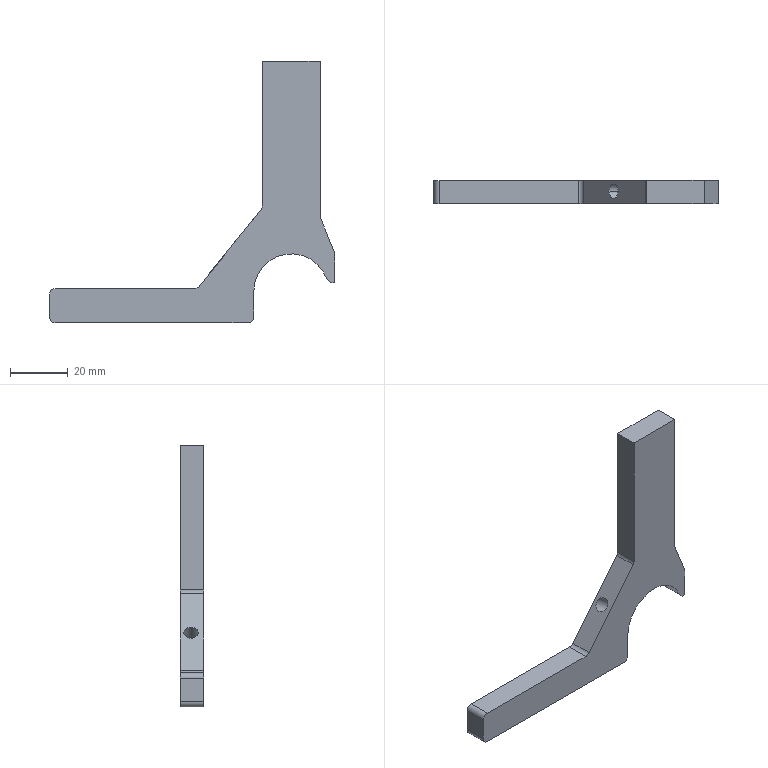Component | SolidWorks | BearingLiftingModule-1_CHEN123-AA-24-1 | 1 solid | 24 faces | box 99 x 8 x 91 mm | volume 20489 mm3 | plane 14 | cylinder 10 | commonest cylinder face diameters 4 x7 5 x2 26.05 x1
STEP:
#1=CARTESIAN_POINT('',(2.27,1.567,1.346));
#2=VERTEX_POINT('',#1);
#3=CARTESIAN_POINT('',(2.37,1.567,1.518));
#4=VERTEX_POINT('',#3);
#5=CARTESIAN_POINT('',(2.27,1.567,1.346));
#6=CARTESIAN_POINT('',(2.27,1.561,1.346));
#7=CARTESIAN_POINT('',(2.27,1.554,1.346));
#8=CARTESIAN_POINT('',(2.271,1.542,1.349));
#9=CARTESIAN_POINT('',(2.272,1.535,1.351));
#10=CARTESIAN_POINT('',(2.274,1.524,1.356));
#11=CARTESIAN_POINT('',(2.275,1.518,1.359));
#12=CARTESIAN_POINT('',(2.278,1.507,1.366));
#13=CARTESIAN_POINT('',(2.279,1.502,1.37));
#14=CARTESIAN_POINT('',(2.283,1.493,1.378));
#15=CARTESIAN_POINT('',(2.285,1.489,1.383));
#16=CARTESIAN_POINT('',(2.289,1.482,1.393));
#17=CARTESIAN_POINT('',(2.291,1.479,1.398));
#18=CARTESIAN_POINT('',(2.299,1.472,1.415));
#19=CARTESIAN_POINT('',(2.305,1.469,1.426));
#20=CARTESIAN_POINT('',(2.315,1.469,1.443));
#21=CARTESIAN_POINT('',(2.318,1.469,1.449));
#22=CARTESIAN_POINT('',(2.325,1.472,1.459));
#23=CARTESIAN_POINT('',(2.329,1.474,1.465));
#24=CARTESIAN_POINT('',(2.335,1.478,1.475));
#25=CARTESIAN_POINT('',(2.339,1.481,1.479));
#26=CARTESIAN_POINT('',(2.345,1.489,1.488));
#27=CARTESIAN_POINT('',(2.348,1.493,1.492));
#28=CARTESIAN_POINT('',(2.357,1.506,1.503));
#29=CARTESIAN_POINT('',(2.361,1.517,1.509));
#30=CARTESIAN_POINT('',(2.366,1.535,1.515));
#31=CARTESIAN_POINT('',(2.368,1.542,1.516));
#32=CARTESIAN_POINT('',(2.369,1.554,1.518));
#33=CARTESIAN_POINT('',(2.37,1.561,1.518));
#34=CARTESIAN_POINT('',(2.37,1.567,1.518));
#35=B_SPLINE_CURVE_WITH_KNOTS('',3,(#5,#6,#7,#8,#9,#10,#11,#12,#13,#14,#15,#16,#17,#18,#19,#20,#21,#22,#23,#24,#25,#26,#27,#28,#29,#30,#31,#32,#33,#34),.UNSPECIFIED.,.F.,.F.,(4,2,2,2,2,2,2,2,2,2,2,2,2,2,4),(0.007885,0.008378,0.008871,0.009363,0.009856,0.01035,0.01084,0.01183,0.01232,0.01281,0.0133,0.0138,0.01478,0.01527,0.01577),.UNSPECIFIED.);
#36=EDGE_CURVE('',#2,#4,#35,.T.);
#37=ORIENTED_EDGE('',*,*,#36,.F.);
#38=CARTESIAN_POINT('',(1.849,1.567,1.687));
#39=VERTEX_POINT('',#38);
#40=CARTESIAN_POINT('',(1.849,1.567,1.687));
#41=DIRECTION('',(-0.7772,0.,0.6292));
#42=VECTOR('',#41,39.37);
#43=LINE('',#40,#42);
#44=EDGE_CURVE('',#2,#39,#43,.T.);
#45=ORIENTED_EDGE('',*,*,#44,.T.);
#46=CARTESIAN_POINT('',(1.973,1.567,1.84));
#47=VERTEX_POINT('',#46);
#48=CARTESIAN_POINT('',(1.911,1.567,1.763));
#49=DIRECTION('',(-0.7772,0.,0.6292));
#50=DIRECTION('',(0.6292,0.,0.7772));
#51=AXIS2_PLACEMENT_3D('',#48,#49,#50);
#52=CIRCLE('',#51,0.09843);
#53=EDGE_CURVE('',#39,#47,#52,.T.);
#54=ORIENTED_EDGE('',*,*,#53,.T.);
#55=CARTESIAN_POINT('',(1.973,1.567,1.84));
#56=DIRECTION('',(-0.7772,0.,0.6292));
#57=VECTOR('',#56,39.37);
#58=LINE('',#55,#57);
#59=EDGE_CURVE('',#4,#47,#58,.T.);
#60=ORIENTED_EDGE('',*,*,#59,.F.);
#61=EDGE_LOOP('',(#37,#45,#54,#60));
#62=FACE_OUTER_BOUND('',#61,.T.);
#63=CARTESIAN_POINT('',(1.911,1.567,1.763));
#64=DIRECTION('',(-0.7772,0.,0.6292));
#65=DIRECTION('',(0.6292,0.,0.7772));
#66=AXIS2_PLACEMENT_3D('',#63,#64,#65);
#67=CYLINDRICAL_SURFACE('',#66,0.09843);
#68=ADVANCED_FACE('',(#62),#67,.F.);
#69=CARTESIAN_POINT('',(2.164,1.713,0.748));
#70=VERTEX_POINT('',#69);
#71=CARTESIAN_POINT('',(-0.4725,1.713,0.748));
#72=VERTEX_POINT('',#71);
#73=CARTESIAN_POINT('',(-0.5512,1.713,0.748));
#74=DIRECTION('',(-1.,0.,0.));
#75=VECTOR('',#74,39.37);
#76=LINE('',#73,#75);
#77=EDGE_CURVE('',#70,#72,#76,.T.);
#78=ORIENTED_EDGE('',*,*,#77,.F.);
#79=CARTESIAN_POINT('',(2.164,1.398,0.748));
#80=VERTEX_POINT('',#79);
#81=CARTESIAN_POINT('',(2.164,1.713,0.748));
#82=DIRECTION('',(0.,-1.,0.));
#83=VECTOR('',#82,39.37);
#84=LINE('',#81,#83);
#85=EDGE_CURVE('',#70,#80,#84,.T.);
#86=ORIENTED_EDGE('',*,*,#85,.T.);
#87=CARTESIAN_POINT('',(-0.4725,1.398,0.748));
#88=VERTEX_POINT('',#87);
#89=CARTESIAN_POINT('',(-0.5512,1.398,0.748));
#90=DIRECTION('',(-1.,0.,0.));
#91=VECTOR('',#90,39.37);
#92=LINE('',#89,#91);
#93=EDGE_CURVE('',#80,#88,#92,.T.);
#94=ORIENTED_EDGE('',*,*,#93,.T.);
#95=CARTESIAN_POINT('',(-0.4725,1.713,0.748));
#96=DIRECTION('',(0.,1.,0.));
#97=VECTOR('',#96,39.37);
#98=LINE('',#95,#97);
#99=EDGE_CURVE('',#88,#72,#98,.T.);
#100=ORIENTED_EDGE('',*,*,#99,.T.);
#101=EDGE_LOOP('',(#78,#86,#94,#100));
#102=FACE_OUTER_BOUND('',#101,.T.);
#103=CARTESIAN_POINT('',(-0.5512,1.713,0.748));
#104=DIRECTION('',(0.,0.,1.));
#105=DIRECTION('',(0.,-1.,0.));
#106=AXIS2_PLACEMENT_3D('',#103,#104,#105);
#107=PLANE('',#106);
#108=ADVANCED_FACE('',(#102),#107,.F.);
#109=CARTESIAN_POINT('',(3.346,1.713,1.695));
#110=VERTEX_POINT('',#109);
#111=CARTESIAN_POINT('',(3.346,1.713,1.299));
#112=VERTEX_POINT('',#111);
#113=CARTESIAN_POINT('',(3.346,1.713,4.331));
#114=DIRECTION('',(0.,0.,-1.));
#115=VECTOR('',#114,39.37);
#116=LINE('',#113,#115);
#117=EDGE_CURVE('',#110,#112,#116,.T.);
#118=ORIENTED_EDGE('',*,*,#117,.F.);
#119=CARTESIAN_POINT('',(3.346,1.398,1.695));
#120=VERTEX_POINT('',#119);
#121=CARTESIAN_POINT('',(3.346,1.713,1.695));
#122=DIRECTION('',(0.,-1.,0.));
#123=VECTOR('',#122,39.37);
#124=LINE('',#121,#123);
#125=EDGE_CURVE('',#110,#120,#124,.T.);
#126=ORIENTED_EDGE('',*,*,#125,.T.);
#127=CARTESIAN_POINT('',(3.346,1.398,1.299));
#128=VERTEX_POINT('',#127);
#129=CARTESIAN_POINT('',(3.346,1.398,4.331));
#130=DIRECTION('',(0.,0.,-1.));
#131=VECTOR('',#130,39.37);
#132=LINE('',#129,#131);
#133=EDGE_CURVE('',#120,#128,#132,.T.);
#134=ORIENTED_EDGE('',*,*,#133,.T.);
#135=CARTESIAN_POINT('',(3.346,1.713,1.299));
#136=DIRECTION('',(0.,1.,0.));
#137=VECTOR('',#136,39.37);
#138=LINE('',#135,#137);
#139=EDGE_CURVE('',#128,#112,#138,.T.);
#140=ORIENTED_EDGE('',*,*,#139,.T.);
#141=EDGE_LOOP('',(#118,#126,#134,#140));
#142=FACE_OUTER_BOUND('',#141,.T.);
#143=CARTESIAN_POINT('',(3.346,1.713,4.331));
#144=DIRECTION('',(-1.,0.,0.));
#145=DIRECTION('',(0.,1.,0.));
#146=AXIS2_PLACEMENT_3D('',#143,#144,#145);
#147=PLANE('',#146);
#148=ADVANCED_FACE('',(#142),#147,.F.);
#149=CARTESIAN_POINT('',(-0.5512,1.713,0.8268));
#150=VERTEX_POINT('',#149);
#151=CARTESIAN_POINT('',(-0.5512,1.713,1.142));
#152=VERTEX_POINT('',#151);
#153=CARTESIAN_POINT('',(-0.5512,1.713,4.331));
#154=DIRECTION('',(0.,0.,1.));
#155=VECTOR('',#154,39.37);
#156=LINE('',#153,#155);
#157=EDGE_CURVE('',#150,#152,#156,.T.);
#158=ORIENTED_EDGE('',*,*,#157,.F.);
#159=CARTESIAN_POINT('',(-0.5512,1.398,0.8268));
#160=VERTEX_POINT('',#159);
#161=CARTESIAN_POINT('',(-0.5512,1.713,0.8268));
#162=DIRECTION('',(0.,-1.,0.));
#163=VECTOR('',#162,39.37);
#164=LINE('',#161,#163);
#165=EDGE_CURVE('',#150,#160,#164,.T.);
#166=ORIENTED_EDGE('',*,*,#165,.T.);
#167=CARTESIAN_POINT('',(-0.5512,1.398,1.142));
#168=VERTEX_POINT('',#167);
#169=CARTESIAN_POINT('',(-0.5512,1.398,4.331));
#170=DIRECTION('',(0.,0.,1.));
#171=VECTOR('',#170,39.37);
#172=LINE('',#169,#171);
#173=EDGE_CURVE('',#160,#168,#172,.T.);
#174=ORIENTED_EDGE('',*,*,#173,.T.);
#175=CARTESIAN_POINT('',(-0.5512,1.713,1.142));
#176=DIRECTION('',(0.,1.,0.));
#177=VECTOR('',#176,39.37);
#178=LINE('',#175,#177);
#179=EDGE_CURVE('',#168,#152,#178,.T.);
#180=ORIENTED_EDGE('',*,*,#179,.T.);
#181=EDGE_LOOP('',(#158,#166,#174,#180));
#182=FACE_OUTER_BOUND('',#181,.T.);
#183=CARTESIAN_POINT('',(-0.5512,1.713,4.331));
#184=DIRECTION('',(1.,0.,0.));
#185=DIRECTION('',(0.,-1.,0.));
#186=AXIS2_PLACEMENT_3D('',#183,#184,#185);
#187=PLANE('',#186);
#188=ADVANCED_FACE('',(#182),#187,.F.);
#189=CARTESIAN_POINT('',(2.362,1.398,4.331));
#190=VERTEX_POINT('',#189);
#191=CARTESIAN_POINT('',(3.15,1.398,4.331));
#192=VERTEX_POINT('',#191);
#193=CARTESIAN_POINT('',(-0.5512,1.398,4.331));
#194=DIRECTION('',(1.,0.,0.));
#195=VECTOR('',#194,39.37);
#196=LINE('',#193,#195);
#197=EDGE_CURVE('',#190,#192,#196,.T.);
#198=ORIENTED_EDGE('',*,*,#197,.T.);
#199=CARTESIAN_POINT('',(3.15,1.713,4.331));
#200=VERTEX_POINT('',#199);
#201=CARTESIAN_POINT('',(3.15,1.398,4.331));
#202=DIRECTION('',(0.,1.,0.));
#203=VECTOR('',#202,39.37);
#204=LINE('',#201,#203);
#205=EDGE_CURVE('',#192,#200,#204,.T.);
#206=ORIENTED_EDGE('',*,*,#205,.T.);
#207=CARTESIAN_POINT('',(2.362,1.713,4.331));
#208=VERTEX_POINT('',#207);
#209=CARTESIAN_POINT('',(-0.5512,1.713,4.331));
#210=DIRECTION('',(1.,0.,0.));
#211=VECTOR('',#210,39.37);
#212=LINE('',#209,#211);
#213=EDGE_CURVE('',#208,#200,#212,.T.);
#214=ORIENTED_EDGE('',*,*,#213,.F.);
#215=CARTESIAN_POINT('',(2.362,1.398,4.331));
#216=DIRECTION('',(0.,1.,0.));
#217=VECTOR('',#216,39.37);
#218=LINE('',#215,#217);
#219=EDGE_CURVE('',#190,#208,#218,.T.);
#220=ORIENTED_EDGE('',*,*,#219,.F.);
#221=EDGE_LOOP('',(#198,#206,#214,#220));
#222=FACE_OUTER_BOUND('',#221,.T.);
#223=CARTESIAN_POINT('',(-0.5512,1.713,4.331));
#224=DIRECTION('',(0.,0.,-1.));
#225=DIRECTION('',(0.,1.,0.));
#226=AXIS2_PLACEMENT_3D('',#223,#224,#225);
#227=PLANE('',#226);
#228=ADVANCED_FACE('',(#222),#227,.F.);
#229=CARTESIAN_POINT('',(3.341,1.713,1.724));
#230=VERTEX_POINT('',#229);
#231=CARTESIAN_POINT('',(3.155,1.713,2.187));
#232=VERTEX_POINT('',#231);
#233=CARTESIAN_POINT('',(3.346,1.713,1.71));
#234=DIRECTION('',(-0.3723,0.,0.9281));
#235=VECTOR('',#234,39.37);
#236=LINE('',#233,#235);
#237=EDGE_CURVE('',#230,#232,#236,.T.);
#238=ORIENTED_EDGE('',*,*,#237,.F.);
#239=CARTESIAN_POINT('',(3.268,1.713,1.695));
#240=DIRECTION('',(0.,1.,0.));
#241=DIRECTION('',(-1.,0.,-0.));
#242=AXIS2_PLACEMENT_3D('',#239,#240,#241);
#243=CIRCLE('',#242,0.07874);
#244=EDGE_CURVE('',#230,#110,#243,.T.);
#245=ORIENTED_EDGE('',*,*,#244,.T.);
#246=ORIENTED_EDGE('',*,*,#117,.T.);
#247=CARTESIAN_POINT('',(3.294,1.713,1.299));
#248=VERTEX_POINT('',#247);
#249=CARTESIAN_POINT('',(2.959,1.713,1.299));
#250=DIRECTION('',(1.,0.,0.));
#251=VECTOR('',#250,39.37);
#252=LINE('',#249,#251);
#253=EDGE_CURVE('',#248,#112,#252,.T.);
#254=ORIENTED_EDGE('',*,*,#253,.F.);
#255=CARTESIAN_POINT('',(3.238,1.713,1.355));
#256=VERTEX_POINT('',#255);
#257=CARTESIAN_POINT('',(3.238,1.713,1.355));
#258=DIRECTION('',(-0.7071,0.,0.7071));
#259=VECTOR('',#258,39.37);
#260=LINE('',#257,#259);
#261=EDGE_CURVE('',#248,#256,#260,.T.);
#262=ORIENTED_EDGE('',*,*,#261,.T.);
#263=CARTESIAN_POINT('',(2.243,1.713,1.181));
#264=VERTEX_POINT('',#263);
#265=CARTESIAN_POINT('',(2.756,1.713,1.181));
#266=DIRECTION('',(0.,1.,0.));
#267=DIRECTION('',(1.,0.,0.));
#268=AXIS2_PLACEMENT_3D('',#265,#266,#267);
#269=CIRCLE('',#268,0.5128);
#270=EDGE_CURVE('',#264,#256,#269,.T.);
#271=ORIENTED_EDGE('',*,*,#270,.F.);
#272=CARTESIAN_POINT('',(2.243,1.713,0.8268));
#273=VERTEX_POINT('',#272);
#274=CARTESIAN_POINT('',(2.243,1.713,1.181));
#275=DIRECTION('',(0.,0.,1.));
#276=VECTOR('',#275,39.37);
#277=LINE('',#274,#276);
#278=EDGE_CURVE('',#273,#264,#277,.T.);
#279=ORIENTED_EDGE('',*,*,#278,.F.);
#280=CARTESIAN_POINT('',(2.164,1.713,0.8268));
#281=DIRECTION('',(0.,1.,0.));
#282=DIRECTION('',(-1.,0.,0.));
#283=AXIS2_PLACEMENT_3D('',#280,#281,#282);
#284=CIRCLE('',#283,0.07874);
#285=EDGE_CURVE('',#273,#70,#284,.T.);
#286=ORIENTED_EDGE('',*,*,#285,.T.);
#287=ORIENTED_EDGE('',*,*,#77,.T.);
#288=CARTESIAN_POINT('',(-0.4725,1.713,0.8268));
#289=DIRECTION('',(0.,1.,0.));
#290=DIRECTION('',(-1.,0.,0.));
#291=AXIS2_PLACEMENT_3D('',#288,#289,#290);
#292=CIRCLE('',#291,0.07874);
#293=EDGE_CURVE('',#72,#150,#292,.T.);
#294=ORIENTED_EDGE('',*,*,#293,.T.);
#295=ORIENTED_EDGE('',*,*,#157,.T.);
#296=CARTESIAN_POINT('',(-0.4725,1.713,1.22));
#297=VERTEX_POINT('',#296);
#298=CARTESIAN_POINT('',(-0.4725,1.713,1.142));
#299=DIRECTION('',(0.,1.,0.));
#300=DIRECTION('',(-1.,0.,0.));
#301=AXIS2_PLACEMENT_3D('',#298,#299,#300);
#302=CIRCLE('',#301,0.07874);
#303=EDGE_CURVE('',#152,#297,#302,.T.);
#304=ORIENTED_EDGE('',*,*,#303,.T.);
#305=CARTESIAN_POINT('',(1.434,1.713,1.22));
#306=VERTEX_POINT('',#305);
#307=CARTESIAN_POINT('',(-0.5512,1.713,1.22));
#308=DIRECTION('',(-1.,0.,0.));
#309=VECTOR('',#308,39.37);
#310=LINE('',#307,#309);
#311=EDGE_CURVE('',#306,#297,#310,.T.);
#312=ORIENTED_EDGE('',*,*,#311,.F.);
#313=CARTESIAN_POINT('',(1.495,1.713,1.25));
#314=VERTEX_POINT('',#313);
#315=CARTESIAN_POINT('',(1.434,1.713,1.299));
#316=DIRECTION('',(0.,-1.,0.));
#317=DIRECTION('',(-1.,0.,0.));
#318=AXIS2_PLACEMENT_3D('',#315,#316,#317);
#319=CIRCLE('',#318,0.07874);
#320=EDGE_CURVE('',#306,#314,#319,.T.);
#321=ORIENTED_EDGE('',*,*,#320,.T.);
#322=CARTESIAN_POINT('',(2.345,1.713,2.299));
#323=VERTEX_POINT('',#322);
#324=CARTESIAN_POINT('',(1.471,1.713,1.22));
#325=DIRECTION('',(-0.6292,0.,-0.7772));
#326=VECTOR('',#325,39.37);
#327=LINE('',#324,#326);
#328=EDGE_CURVE('',#323,#314,#327,.T.);
#329=ORIENTED_EDGE('',*,*,#328,.F.);
#330=CARTESIAN_POINT('',(2.362,1.713,2.349));
#331=VERTEX_POINT('',#330);
#332=CARTESIAN_POINT('',(2.283,1.713,2.349));
#333=DIRECTION('',(0.,-1.,0.));
#334=DIRECTION('',(-1.,0.,0.));
#335=AXIS2_PLACEMENT_3D('',#332,#333,#334);
#336=CIRCLE('',#335,0.07874);
#337=EDGE_CURVE('',#323,#331,#336,.T.);
#338=ORIENTED_EDGE('',*,*,#337,.T.);
#339=CARTESIAN_POINT('',(2.362,1.713,2.321));
#340=DIRECTION('',(-0.,0.,-1.));
#341=VECTOR('',#340,39.37);
#342=LINE('',#339,#341);
#343=EDGE_CURVE('',#208,#331,#342,.T.);
#344=ORIENTED_EDGE('',*,*,#343,.F.);
#345=ORIENTED_EDGE('',*,*,#213,.T.);
#346=CARTESIAN_POINT('',(3.15,1.713,2.216));
#347=VERTEX_POINT('',#346);
#348=CARTESIAN_POINT('',(3.15,1.713,4.331));
#349=DIRECTION('',(0.,0.,1.));
#350=VECTOR('',#349,39.37);
#351=LINE('',#348,#350);
#352=EDGE_CURVE('',#347,#200,#351,.T.);
#353=ORIENTED_EDGE('',*,*,#352,.F.);
#354=CARTESIAN_POINT('',(3.228,1.713,2.216));
#355=DIRECTION('',(0.,-1.,0.));
#356=DIRECTION('',(-1.,0.,0.));
#357=AXIS2_PLACEMENT_3D('',#354,#355,#356);
#358=CIRCLE('',#357,0.07874);
#359=EDGE_CURVE('',#347,#232,#358,.T.);
#360=ORIENTED_EDGE('',*,*,#359,.T.);
#361=EDGE_LOOP('',(#238,#245,#246,#254,#262,#271,#279,#286,#287,#294,#295,#304,#312,#321,#329,#338,#344,#345,#353,#360));
#362=FACE_OUTER_BOUND('',#361,.T.);
#363=CARTESIAN_POINT('',(1.398,1.713,2.539));
#364=DIRECTION('',(0.,-1.,0.));
#365=DIRECTION('',(-1.,0.,0.));
#366=AXIS2_PLACEMENT_3D('',#363,#364,#365);
#367=PLANE('',#366);
#368=ADVANCED_FACE('',(#362),#367,.F.);
#369=ORIENTED_EDGE('',*,*,#133,.F.);
#370=CARTESIAN_POINT('',(3.341,1.398,1.724));
#371=VERTEX_POINT('',#370);
#372=CARTESIAN_POINT('',(3.268,1.398,1.695));
#373=DIRECTION('',(0.,-1.,0.));
#374=DIRECTION('',(-1.,0.,0.));
#375=AXIS2_PLACEMENT_3D('',#372,#373,#374);
#376=CIRCLE('',#375,0.07874);
#377=EDGE_CURVE('',#120,#371,#376,.T.);
#378=ORIENTED_EDGE('',*,*,#377,.T.);
#379=CARTESIAN_POINT('',(3.155,1.398,2.187));
#380=VERTEX_POINT('',#379);
#381=CARTESIAN_POINT('',(3.346,1.398,1.71));
#382=DIRECTION('',(-0.3723,0.,0.9281));
#383=VECTOR('',#382,39.37);
#384=LINE('',#381,#383);
#385=EDGE_CURVE('',#371,#380,#384,.T.);
#386=ORIENTED_EDGE('',*,*,#385,.T.);
#387=CARTESIAN_POINT('',(3.15,1.398,2.216));
#388=VERTEX_POINT('',#387);
#389=CARTESIAN_POINT('',(3.228,1.398,2.216));
#390=DIRECTION('',(0.,1.,0.));
#391=DIRECTION('',(-1.,0.,-0.));
#392=AXIS2_PLACEMENT_3D('',#389,#390,#391);
#393=CIRCLE('',#392,0.07874);
#394=EDGE_CURVE('',#380,#388,#393,.T.);
#395=ORIENTED_EDGE('',*,*,#394,.T.);
#396=CARTESIAN_POINT('',(3.15,1.398,4.331));
#397=DIRECTION('',(0.,0.,1.));
#398=VECTOR('',#397,39.37);
#399=LINE('',#396,#398);
#400=EDGE_CURVE('',#388,#192,#399,.T.);
#401=ORIENTED_EDGE('',*,*,#400,.T.);
#402=ORIENTED_EDGE('',*,*,#197,.F.);
#403=CARTESIAN_POINT('',(2.362,1.398,2.349));
#404=VERTEX_POINT('',#403);
#405=CARTESIAN_POINT('',(2.362,1.398,2.321));
#406=DIRECTION('',(-0.,0.,-1.));
#407=VECTOR('',#406,39.37);
#408=LINE('',#405,#407);
#409=EDGE_CURVE('',#190,#404,#408,.T.);
#410=ORIENTED_EDGE('',*,*,#409,.T.);
#411=CARTESIAN_POINT('',(2.345,1.398,2.299));
#412=VERTEX_POINT('',#411);
#413=CARTESIAN_POINT('',(2.283,1.398,2.349));
#414=DIRECTION('',(0.,1.,0.));
#415=DIRECTION('',(-1.,0.,0.));
#416=AXIS2_PLACEMENT_3D('',#413,#414,#415);
#417=CIRCLE('',#416,0.07874);
#418=EDGE_CURVE('',#404,#412,#417,.T.);
#419=ORIENTED_EDGE('',*,*,#418,.T.);
#420=CARTESIAN_POINT('',(1.495,1.398,1.25));
#421=VERTEX_POINT('',#420);
#422=CARTESIAN_POINT('',(1.471,1.398,1.22));
#423=DIRECTION('',(-0.6292,0.,-0.7772));
#424=VECTOR('',#423,39.37);
#425=LINE('',#422,#424);
#426=EDGE_CURVE('',#412,#421,#425,.T.);
#427=ORIENTED_EDGE('',*,*,#426,.T.);
#428=CARTESIAN_POINT('',(1.434,1.398,1.22));
#429=VERTEX_POINT('',#428);
#430=CARTESIAN_POINT('',(1.434,1.398,1.299));
#431=DIRECTION('',(0.,1.,0.));
#432=DIRECTION('',(-1.,0.,0.));
#433=AXIS2_PLACEMENT_3D('',#430,#431,#432);
#434=CIRCLE('',#433,0.07874);
#435=EDGE_CURVE('',#421,#429,#434,.T.);
#436=ORIENTED_EDGE('',*,*,#435,.T.);
#437=CARTESIAN_POINT('',(-0.4725,1.398,1.22));
#438=VERTEX_POINT('',#437);
#439=CARTESIAN_POINT('',(-0.5512,1.398,1.22));
#440=DIRECTION('',(-1.,0.,0.));
#441=VECTOR('',#440,39.37);
#442=LINE('',#439,#441);
#443=EDGE_CURVE('',#429,#438,#442,.T.);
#444=ORIENTED_EDGE('',*,*,#443,.T.);
#445=CARTESIAN_POINT('',(-0.4725,1.398,1.142));
#446=DIRECTION('',(0.,-1.,0.));
#447=DIRECTION('',(-1.,0.,0.));
#448=AXIS2_PLACEMENT_3D('',#445,#446,#447);
#449=CIRCLE('',#448,0.07874);
#450=EDGE_CURVE('',#438,#168,#449,.T.);
#451=ORIENTED_EDGE('',*,*,#450,.T.);
#452=ORIENTED_EDGE('',*,*,#173,.F.);
#453=CARTESIAN_POINT('',(-0.4725,1.398,0.8268));
#454=DIRECTION('',(0.,-1.,0.));
#455=DIRECTION('',(-1.,0.,0.));
#456=AXIS2_PLACEMENT_3D('',#453,#454,#455);
#457=CIRCLE('',#456,0.07874);
#458=EDGE_CURVE('',#160,#88,#457,.T.);
#459=ORIENTED_EDGE('',*,*,#458,.T.);
#460=ORIENTED_EDGE('',*,*,#93,.F.);
#461=CARTESIAN_POINT('',(2.243,1.398,0.8268));
#462=VERTEX_POINT('',#461);
#463=CARTESIAN_POINT('',(2.164,1.398,0.8268));
#464=DIRECTION('',(0.,-1.,0.));
#465=DIRECTION('',(-1.,0.,0.));
#466=AXIS2_PLACEMENT_3D('',#463,#464,#465);
#467=CIRCLE('',#466,0.07874);
#468=EDGE_CURVE('',#80,#462,#467,.T.);
#469=ORIENTED_EDGE('',*,*,#468,.T.);
#470=CARTESIAN_POINT('',(2.243,1.398,1.181));
#471=VERTEX_POINT('',#470);
#472=CARTESIAN_POINT('',(2.243,1.398,2.539));
#473=DIRECTION('',(0.,0.,-1.));
#474=VECTOR('',#473,39.37);
#475=LINE('',#472,#474);
#476=EDGE_CURVE('',#471,#462,#475,.T.);
#477=ORIENTED_EDGE('',*,*,#476,.F.);
#478=CARTESIAN_POINT('',(3.238,1.398,1.355));
#479=VERTEX_POINT('',#478);
#480=CARTESIAN_POINT('',(2.756,1.398,1.181));
#481=DIRECTION('',(0.,1.,0.));
#482=DIRECTION('',(1.,0.,0.));
#483=AXIS2_PLACEMENT_3D('',#480,#481,#482);
#484=CIRCLE('',#483,0.5128);
#485=EDGE_CURVE('',#471,#479,#484,.T.);
#486=ORIENTED_EDGE('',*,*,#485,.T.);
#487=CARTESIAN_POINT('',(3.294,1.398,1.299));
#488=VERTEX_POINT('',#487);
#489=CARTESIAN_POINT('',(1.726,1.398,2.868));
#490=DIRECTION('',(0.7071,0.,-0.7071));
#491=VECTOR('',#490,39.37);
#492=LINE('',#489,#491);
#493=EDGE_CURVE('',#479,#488,#492,.T.);
#494=ORIENTED_EDGE('',*,*,#493,.T.);
#495=CARTESIAN_POINT('',(2.959,1.398,1.299));
#496=DIRECTION('',(1.,0.,0.));
#497=VECTOR('',#496,39.37);
#498=LINE('',#495,#497);
#499=EDGE_CURVE('',#488,#128,#498,.T.);
#500=ORIENTED_EDGE('',*,*,#499,.T.);
#501=EDGE_LOOP('',(#369,#378,#386,#395,#401,#402,#410,#419,#427,#436,#444,#451,#452,#459,#460,#469,#477,#486,#494,#500));
#502=FACE_OUTER_BOUND('',#501,.T.);
#503=CARTESIAN_POINT('',(1.398,1.398,2.539));
#504=DIRECTION('',(0.,-1.,0.));
#505=DIRECTION('',(-1.,0.,0.));
#506=AXIS2_PLACEMENT_3D('',#503,#504,#505);
#507=PLANE('',#506);
#508=ADVANCED_FACE('',(#502),#507,.T.);
#509=ORIENTED_EDGE('',*,*,#443,.F.);
#510=CARTESIAN_POINT('',(1.434,1.713,1.22));
#511=DIRECTION('',(0.,1.,0.));
#512=VECTOR('',#511,39.37);
#513=LINE('',#510,#512);
#514=EDGE_CURVE('',#429,#306,#513,.T.);
#515=ORIENTED_EDGE('',*,*,#514,.T.);
#516=ORIENTED_EDGE('',*,*,#311,.T.);
#517=CARTESIAN_POINT('',(-0.4725,1.398,1.22));
#518=DIRECTION('',(0.,-1.,0.));
#519=VECTOR('',#518,39.37);
#520=LINE('',#517,#519);
#521=EDGE_CURVE('',#297,#438,#520,.T.);
#522=ORIENTED_EDGE('',*,*,#521,.T.);
#523=EDGE_LOOP('',(#509,#515,#516,#522));
#524=FACE_OUTER_BOUND('',#523,.T.);
#525=CARTESIAN_POINT('',(-0.5512,1.398,1.22));
#526=DIRECTION('',(0.,0.,-1.));
#527=DIRECTION('',(0.,1.,0.));
#528=AXIS2_PLACEMENT_3D('',#525,#526,#527);
#529=PLANE('',#528);
#530=ADVANCED_FACE('',(#524),#529,.F.);
#531=CARTESIAN_POINT('',(1.911,1.567,1.763));
#532=DIRECTION('',(-0.7772,0.,0.6292));
#533=DIRECTION('',(0.6292,0.,0.7772));
#534=AXIS2_PLACEMENT_3D('',#531,#532,#533);
#535=CIRCLE('',#534,0.09843);
#536=EDGE_CURVE('',#47,#39,#535,.T.);
#537=ORIENTED_EDGE('',*,*,#536,.F.);
#538=ORIENTED_EDGE('',*,*,#53,.F.);
#539=EDGE_LOOP('',(#537,#538));
#540=FACE_BOUND('',#539,.T.);
#541=ORIENTED_EDGE('',*,*,#328,.T.);
#542=CARTESIAN_POINT('',(1.495,1.398,1.25));
#543=DIRECTION('',(0.,-1.,0.));
#544=VECTOR('',#543,39.37);
#545=LINE('',#542,#544);
#546=EDGE_CURVE('',#314,#421,#545,.T.);
#547=ORIENTED_EDGE('',*,*,#546,.T.);
#548=ORIENTED_EDGE('',*,*,#426,.F.);
#549=CARTESIAN_POINT('',(2.345,1.713,2.299));
#550=DIRECTION('',(0.,1.,0.));
#551=VECTOR('',#550,39.37);
#552=LINE('',#549,#551);
#553=EDGE_CURVE('',#412,#323,#552,.T.);
#554=ORIENTED_EDGE('',*,*,#553,.T.);
#555=EDGE_LOOP('',(#541,#547,#548,#554));
#556=FACE_OUTER_BOUND('',#555,.T.);
#557=CARTESIAN_POINT('',(1.471,1.398,1.22));
#558=DIRECTION('',(0.7772,0.,-0.6292));
#559=DIRECTION('',(-0.6292,0.,-0.7772));
#560=AXIS2_PLACEMENT_3D('',#557,#558,#559);
#561=PLANE('',#560);
#562=ADVANCED_FACE('',(#540,#556),#561,.F.);
#563=ORIENTED_EDGE('',*,*,#343,.T.);
#564=CARTESIAN_POINT('',(2.362,1.398,2.349));
#565=DIRECTION('',(0.,-1.,0.));
#566=VECTOR('',#565,39.37);
#567=LINE('',#564,#566);
#568=EDGE_CURVE('',#331,#404,#567,.T.);
#569=ORIENTED_EDGE('',*,*,#568,.T.);
#570=ORIENTED_EDGE('',*,*,#409,.F.);
#571=ORIENTED_EDGE('',*,*,#219,.T.);
#572=EDGE_LOOP('',(#563,#569,#570,#571));
#573=FACE_OUTER_BOUND('',#572,.T.);
#574=CARTESIAN_POINT('',(2.362,1.398,2.321));
#575=DIRECTION('',(1.,0.,-0.));
#576=DIRECTION('',(-0.,0.,-1.));
#577=AXIS2_PLACEMENT_3D('',#574,#575,#576);
#578=PLANE('',#577);
#579=ADVANCED_FACE('',(#573),#578,.F.);
#580=ORIENTED_EDGE('',*,*,#476,.T.);
#581=CARTESIAN_POINT('',(2.243,1.398,0.8268));
#582=DIRECTION('',(0.,1.,0.));
#583=VECTOR('',#582,39.37);
#584=LINE('',#581,#583);
#585=EDGE_CURVE('',#462,#273,#584,.T.);
#586=ORIENTED_EDGE('',*,*,#585,.T.);
#587=ORIENTED_EDGE('',*,*,#278,.T.);
#588=CARTESIAN_POINT('',(2.243,1.398,1.181));
#589=DIRECTION('',(0.,1.,0.));
#590=VECTOR('',#589,39.37);
#591=LINE('',#588,#590);
#592=EDGE_CURVE('',#471,#264,#591,.T.);
#593=ORIENTED_EDGE('',*,*,#592,.F.);
#594=EDGE_LOOP('',(#580,#586,#587,#593));
#595=FACE_OUTER_BOUND('',#594,.T.);
#596=CARTESIAN_POINT('',(2.243,1.398,1.181));
#597=DIRECTION('',(-1.,0.,0.));
#598=DIRECTION('',(0.,1.,0.));
#599=AXIS2_PLACEMENT_3D('',#596,#597,#598);
#600=PLANE('',#599);
#601=ADVANCED_FACE('',(#595),#600,.F.);
#602=CARTESIAN_POINT('',(2.37,1.567,1.518));
#603=CARTESIAN_POINT('',(2.37,1.574,1.518));
#604=CARTESIAN_POINT('',(2.369,1.58,1.518));
#605=CARTESIAN_POINT('',(2.368,1.593,1.516));
#606=CARTESIAN_POINT('',(2.366,1.599,1.515));
#607=CARTESIAN_POINT('',(2.363,1.611,1.511));
#608=CARTESIAN_POINT('',(2.361,1.617,1.508));
#609=CARTESIAN_POINT('',(2.357,1.628,1.503));
#610=CARTESIAN_POINT('',(2.354,1.633,1.499));
#611=CARTESIAN_POINT('',(2.348,1.642,1.492));
#612=CARTESIAN_POINT('',(2.345,1.646,1.488));
#613=CARTESIAN_POINT('',(2.339,1.653,1.479));
#614=CARTESIAN_POINT('',(2.335,1.656,1.475));
#615=CARTESIAN_POINT('',(2.329,1.661,1.465));
#616=CARTESIAN_POINT('',(2.325,1.663,1.459));
#617=CARTESIAN_POINT('',(2.318,1.665,1.449));
#618=CARTESIAN_POINT('',(2.315,1.666,1.443));
#619=CARTESIAN_POINT('',(2.309,1.666,1.432));
#620=CARTESIAN_POINT('',(2.305,1.665,1.426));
#621=CARTESIAN_POINT('',(2.299,1.662,1.415));
#622=CARTESIAN_POINT('',(2.297,1.661,1.409));
#623=CARTESIAN_POINT('',(2.291,1.656,1.398));
#624=CARTESIAN_POINT('',(2.289,1.653,1.393));
#625=CARTESIAN_POINT('',(2.285,1.645,1.383));
#626=CARTESIAN_POINT('',(2.283,1.641,1.379));
#627=CARTESIAN_POINT('',(2.279,1.632,1.37));
#628=CARTESIAN_POINT('',(2.278,1.627,1.366));
#629=CARTESIAN_POINT('',(2.275,1.617,1.359));
#630=CARTESIAN_POINT('',(2.274,1.611,1.356));
#631=CARTESIAN_POINT('',(2.272,1.599,1.351));
#632=CARTESIAN_POINT('',(2.271,1.593,1.349));
#633=CARTESIAN_POINT('',(2.27,1.58,1.346));
#634=CARTESIAN_POINT('',(2.27,1.574,1.346));
#635=CARTESIAN_POINT('',(2.27,1.567,1.346));
#636=B_SPLINE_CURVE_WITH_KNOTS('',3,(#602,#603,#604,#605,#606,#607,#608,#609,#610,#611,#612,#613,#614,#615,#616,#617,#618,#619,#620,#621,#622,#623,#624,#625,#626,#627,#628,#629,#630,#631,#632,#633,#634,#635),.UNSPECIFIED.,.F.,.F.,(4,2,2,2,2,2,2,2,2,2,2,2,2,2,2,2,4),(0.,0.0004928,0.0009857,0.001479,0.001971,0.002464,0.002957,0.00345,0.003943,0.004436,0.004928,0.005421,0.005914,0.006407,0.0069,0.007393,0.007885),.UNSPECIFIED.);
#637=EDGE_CURVE('',#4,#2,#636,.T.);
#638=ORIENTED_EDGE('',*,*,#637,.T.);
#639=ORIENTED_EDGE('',*,*,#36,.T.);
#640=EDGE_LOOP('',(#638,#639));
#641=FACE_BOUND('',#640,.T.);
#642=ORIENTED_EDGE('',*,*,#270,.T.);
#643=CARTESIAN_POINT('',(3.238,1.398,1.355));
#644=DIRECTION('',(0.,-1.,0.));
#645=VECTOR('',#644,39.37);
#646=LINE('',#643,#645);
#647=EDGE_CURVE('',#256,#479,#646,.T.);
#648=ORIENTED_EDGE('',*,*,#647,.T.);
#649=ORIENTED_EDGE('',*,*,#485,.F.);
#650=ORIENTED_EDGE('',*,*,#592,.T.);
#651=EDGE_LOOP('',(#642,#648,#649,#650));
#652=FACE_OUTER_BOUND('',#651,.T.);
#653=CARTESIAN_POINT('',(2.756,1.398,1.181));
#654=DIRECTION('',(0.,1.,0.));
#655=DIRECTION('',(1.,0.,0.));
#656=AXIS2_PLACEMENT_3D('',#653,#654,#655);
#657=CYLINDRICAL_SURFACE('',#656,0.5128);
#658=ADVANCED_FACE('',(#641,#652),#657,.F.);
#659=ORIENTED_EDGE('',*,*,#499,.F.);
#660=CARTESIAN_POINT('',(3.294,1.398,1.299));
#661=DIRECTION('',(0.,1.,0.));
#662=VECTOR('',#661,39.37);
#663=LINE('',#660,#662);
#664=EDGE_CURVE('',#488,#248,#663,.T.);
#665=ORIENTED_EDGE('',*,*,#664,.T.);
#666=ORIENTED_EDGE('',*,*,#253,.T.);
#667=ORIENTED_EDGE('',*,*,#139,.F.);
#668=EDGE_LOOP('',(#659,#665,#666,#667));
#669=FACE_OUTER_BOUND('',#668,.T.);
#670=CARTESIAN_POINT('',(2.959,1.398,1.299));
#671=DIRECTION('',(0.,0.,1.));
#672=DIRECTION('',(0.,-1.,0.));
#673=AXIS2_PLACEMENT_3D('',#670,#671,#672);
#674=PLANE('',#673);
#675=ADVANCED_FACE('',(#669),#674,.F.);
#676=ORIENTED_EDGE('',*,*,#261,.F.);
#677=ORIENTED_EDGE('',*,*,#664,.F.);
#678=ORIENTED_EDGE('',*,*,#493,.F.);
#679=ORIENTED_EDGE('',*,*,#647,.F.);
#680=EDGE_LOOP('',(#676,#677,#678,#679));
#681=FACE_OUTER_BOUND('',#680,.T.);
#682=CARTESIAN_POINT('',(3.238,1.398,1.355));
#683=DIRECTION('',(-0.7071,0.,-0.7071));
#684=DIRECTION('',(0.,1.,0.));
#685=AXIS2_PLACEMENT_3D('',#682,#683,#684);
#686=PLANE('',#685);
#687=ADVANCED_FACE('',(#681),#686,.T.);
#688=ORIENTED_EDGE('',*,*,#400,.F.);
#689=CARTESIAN_POINT('',(3.15,1.713,2.216));
#690=DIRECTION('',(0.,1.,0.));
#691=VECTOR('',#690,39.37);
#692=LINE('',#689,#691);
#693=EDGE_CURVE('',#388,#347,#692,.T.);
#694=ORIENTED_EDGE('',*,*,#693,.T.);
#695=ORIENTED_EDGE('',*,*,#352,.T.);
#696=ORIENTED_EDGE('',*,*,#205,.F.);
#697=EDGE_LOOP('',(#688,#694,#695,#696));
#698=FACE_OUTER_BOUND('',#697,.T.);
#699=CARTESIAN_POINT('',(3.15,1.398,4.331));
#700=DIRECTION('',(-1.,0.,0.));
#701=DIRECTION('',(0.,1.,0.));
#702=AXIS2_PLACEMENT_3D('',#699,#700,#701);
#703=PLANE('',#702);
#704=ADVANCED_FACE('',(#698),#703,.F.);
#705=ORIENTED_EDGE('',*,*,#237,.T.);
#706=CARTESIAN_POINT('',(3.155,1.398,2.187));
#707=DIRECTION('',(0.,-1.,0.));
#708=VECTOR('',#707,39.37);
#709=LINE('',#706,#708);
#710=EDGE_CURVE('',#232,#380,#709,.T.);
#711=ORIENTED_EDGE('',*,*,#710,.T.);
#712=ORIENTED_EDGE('',*,*,#385,.F.);
#713=CARTESIAN_POINT('',(3.341,1.398,1.724));
#714=DIRECTION('',(0.,1.,0.));
#715=VECTOR('',#714,39.37);
#716=LINE('',#713,#715);
#717=EDGE_CURVE('',#371,#230,#716,.T.);
#718=ORIENTED_EDGE('',*,*,#717,.T.);
#719=EDGE_LOOP('',(#705,#711,#712,#718));
#720=FACE_OUTER_BOUND('',#719,.T.);
#721=CARTESIAN_POINT('',(3.346,1.398,1.71));
#722=DIRECTION('',(-0.9281,0.,-0.3723));
#723=DIRECTION('',(-0.3723,0.,0.9281));
#724=AXIS2_PLACEMENT_3D('',#721,#722,#723);
#725=PLANE('',#724);
#726=ADVANCED_FACE('',(#720),#725,.F.);
#727=ORIENTED_EDGE('',*,*,#394,.F.);
#728=ORIENTED_EDGE('',*,*,#710,.F.);
#729=ORIENTED_EDGE('',*,*,#359,.F.);
#730=ORIENTED_EDGE('',*,*,#693,.F.);
#731=EDGE_LOOP('',(#727,#728,#729,#730));
#732=FACE_OUTER_BOUND('',#731,.T.);
#733=CARTESIAN_POINT('',(3.228,1.398,2.216));
#734=DIRECTION('',(0.,-1.,0.));
#735=DIRECTION('',(-1.,0.,0.));
#736=AXIS2_PLACEMENT_3D('',#733,#734,#735);
#737=CYLINDRICAL_SURFACE('',#736,0.07874);
#738=ADVANCED_FACE('',(#732),#737,.F.);
#739=ORIENTED_EDGE('',*,*,#377,.F.);
#740=ORIENTED_EDGE('',*,*,#125,.F.);
#741=ORIENTED_EDGE('',*,*,#244,.F.);
#742=ORIENTED_EDGE('',*,*,#717,.F.);
#743=EDGE_LOOP('',(#739,#740,#741,#742));
#744=FACE_OUTER_BOUND('',#743,.T.);
#745=CARTESIAN_POINT('',(3.268,1.398,1.695));
#746=DIRECTION('',(0.,1.,0.));
#747=DIRECTION('',(1.,0.,0.));
#748=AXIS2_PLACEMENT_3D('',#745,#746,#747);
#749=CYLINDRICAL_SURFACE('',#748,0.07874);
#750=ADVANCED_FACE('',(#744),#749,.T.);
#751=ORIENTED_EDGE('',*,*,#285,.F.);
#752=ORIENTED_EDGE('',*,*,#585,.F.);
#753=ORIENTED_EDGE('',*,*,#468,.F.);
#754=ORIENTED_EDGE('',*,*,#85,.F.);
#755=EDGE_LOOP('',(#751,#752,#753,#754));
#756=FACE_OUTER_BOUND('',#755,.T.);
#757=CARTESIAN_POINT('',(2.164,1.713,0.8268));
#758=DIRECTION('',(0.,-1.,0.));
#759=DIRECTION('',(-1.,0.,0.));
#760=AXIS2_PLACEMENT_3D('',#757,#758,#759);
#761=CYLINDRICAL_SURFACE('',#760,0.07874);
#762=ADVANCED_FACE('',(#756),#761,.T.);
#763=ORIENTED_EDGE('',*,*,#293,.F.);
#764=ORIENTED_EDGE('',*,*,#99,.F.);
#765=ORIENTED_EDGE('',*,*,#458,.F.);
#766=ORIENTED_EDGE('',*,*,#165,.F.);
#767=EDGE_LOOP('',(#763,#764,#765,#766));
#768=FACE_OUTER_BOUND('',#767,.T.);
#769=CARTESIAN_POINT('',(-0.4725,1.713,0.8268));
#770=DIRECTION('',(0.,-1.,0.));
#771=DIRECTION('',(-1.,0.,0.));
#772=AXIS2_PLACEMENT_3D('',#769,#770,#771);
#773=CYLINDRICAL_SURFACE('',#772,0.07874);
#774=ADVANCED_FACE('',(#768),#773,.T.);
#775=ORIENTED_EDGE('',*,*,#435,.F.);
#776=ORIENTED_EDGE('',*,*,#546,.F.);
#777=ORIENTED_EDGE('',*,*,#320,.F.);
#778=ORIENTED_EDGE('',*,*,#514,.F.);
#779=EDGE_LOOP('',(#775,#776,#777,#778));
#780=FACE_OUTER_BOUND('',#779,.T.);
#781=CARTESIAN_POINT('',(1.434,1.398,1.299));
#782=DIRECTION('',(0.,-1.,0.));
#783=DIRECTION('',(-1.,0.,0.));
#784=AXIS2_PLACEMENT_3D('',#781,#782,#783);
#785=CYLINDRICAL_SURFACE('',#784,0.07874);
#786=ADVANCED_FACE('',(#780),#785,.F.);
#787=ORIENTED_EDGE('',*,*,#418,.F.);
#788=ORIENTED_EDGE('',*,*,#568,.F.);
#789=ORIENTED_EDGE('',*,*,#337,.F.);
#790=ORIENTED_EDGE('',*,*,#553,.F.);
#791=EDGE_LOOP('',(#787,#788,#789,#790));
#792=FACE_OUTER_BOUND('',#791,.T.);
#793=CARTESIAN_POINT('',(2.283,1.398,2.349));
#794=DIRECTION('',(0.,-1.,0.));
#795=DIRECTION('',(-1.,0.,0.));
#796=AXIS2_PLACEMENT_3D('',#793,#794,#795);
#797=CYLINDRICAL_SURFACE('',#796,0.07874);
#798=ADVANCED_FACE('',(#792),#797,.F.);
#799=ORIENTED_EDGE('',*,*,#450,.F.);
#800=ORIENTED_EDGE('',*,*,#521,.F.);
#801=ORIENTED_EDGE('',*,*,#303,.F.);
#802=ORIENTED_EDGE('',*,*,#179,.F.);
#803=EDGE_LOOP('',(#799,#800,#801,#802));
#804=FACE_OUTER_BOUND('',#803,.T.);
#805=CARTESIAN_POINT('',(-0.4725,1.713,1.142));
#806=DIRECTION('',(0.,1.,0.));
#807=DIRECTION('',(1.,0.,0.));
#808=AXIS2_PLACEMENT_3D('',#805,#806,#807);
#809=CYLINDRICAL_SURFACE('',#808,0.07874);
#810=ADVANCED_FACE('',(#804),#809,.T.);
#811=ORIENTED_EDGE('',*,*,#44,.F.);
#812=ORIENTED_EDGE('',*,*,#637,.F.);
#813=ORIENTED_EDGE('',*,*,#59,.T.);
#814=ORIENTED_EDGE('',*,*,#536,.T.);
#815=EDGE_LOOP('',(#811,#812,#813,#814));
#816=FACE_OUTER_BOUND('',#815,.T.);
#817=CARTESIAN_POINT('',(1.911,1.567,1.763));
#818=DIRECTION('',(-0.7772,0.,0.6292));
#819=DIRECTION('',(0.6292,0.,0.7772));
#820=AXIS2_PLACEMENT_3D('',#817,#818,#819);
#821=CYLINDRICAL_SURFACE('',#820,0.09843);
#822=ADVANCED_FACE('',(#816),#821,.F.);
#823=CLOSED_SHELL('',(#68,#108,#148,#188,#228,#368,#508,#530,#562,#579,#601,#658,#675,#687,#704,#726,#738,#750,#762,#774,#786,#798,#810,#822));
#824=MANIFOLD_SOLID_BREP('',#823);
#825=CARTESIAN_POINT('',(0.,0.,0.));
#826=DIRECTION('',(0.,0.,1.));
#827=DIRECTION('',(1.,0.,0.));
#828=AXIS2_PLACEMENT_3D('',#825,#826,#827);
#829=(LENGTH_UNIT()NAMED_UNIT(*)SI_UNIT($,.METRE.));
#830=LENGTH_MEASURE_WITH_UNIT(LENGTH_MEASURE(0.0254),#829);
#831=DIMENSIONAL_EXPONENTS(1.,0.,0.,0.,0.,0.,0.);
#832=(CONVERSION_BASED_UNIT('',#830)LENGTH_UNIT()NAMED_UNIT(#831));
#833=UNCERTAINTY_MEASURE_WITH_UNIT(LENGTH_MEASURE(0.00001),#832,'','');
#834=(NAMED_UNIT(*)PLANE_ANGLE_UNIT()SI_UNIT($,.RADIAN.));
#835=(NAMED_UNIT(*)SI_UNIT($,.STERADIAN.)SOLID_ANGLE_UNIT());
#836=(GEOMETRIC_REPRESENTATION_CONTEXT(3)GLOBAL_UNCERTAINTY_ASSIGNED_CONTEXT((#833))GLOBAL_UNIT_ASSIGNED_CONTEXT((#832,#834,#835))REPRESENTATION_CONTEXT('',''));
#837=ADVANCED_BREP_SHAPE_REPRESENTATION('',(#824,#828),#836);
#838=COLOUR_RGB('',0.7922,0.8196,0.9333);
#839=FILL_AREA_STYLE_COLOUR('',#838);
#840=FILL_AREA_STYLE('',(#839));
#841=SURFACE_STYLE_FILL_AREA(#840);
#842=SURFACE_SIDE_STYLE('',(#841));
#843=SURFACE_STYLE_USAGE(.BOTH.,#842);
#844=PRESENTATION_STYLE_ASSIGNMENT((#843));
#845=STYLED_ITEM('',(#844),#824);
#846=(LENGTH_UNIT()NAMED_UNIT(*)SI_UNIT($,.METRE.));
#847=LENGTH_MEASURE_WITH_UNIT(LENGTH_MEASURE(0.0254),#846);
#848=DIMENSIONAL_EXPONENTS(1.,0.,0.,0.,0.,0.,0.);
#849=(CONVERSION_BASED_UNIT('',#847)LENGTH_UNIT()NAMED_UNIT(#848));
#850=UNCERTAINTY_MEASURE_WITH_UNIT(LENGTH_MEASURE(0.00001),#849,'','');
#851=(NAMED_UNIT(*)PLANE_ANGLE_UNIT()SI_UNIT($,.RADIAN.));
#852=(NAMED_UNIT(*)SI_UNIT($,.STERADIAN.)SOLID_ANGLE_UNIT());
#853=(GEOMETRIC_REPRESENTATION_CONTEXT(3)GLOBAL_UNCERTAINTY_ASSIGNED_CONTEXT((#850))GLOBAL_UNIT_ASSIGNED_CONTEXT((#849,#851,#852))REPRESENTATION_CONTEXT('',''));
#854=MECHANICAL_DESIGN_GEOMETRIC_PRESENTATION_REPRESENTATION('',(#845),#853);
#855=PRESENTATION_LAYER_ASSIGNMENT('','',(#845));